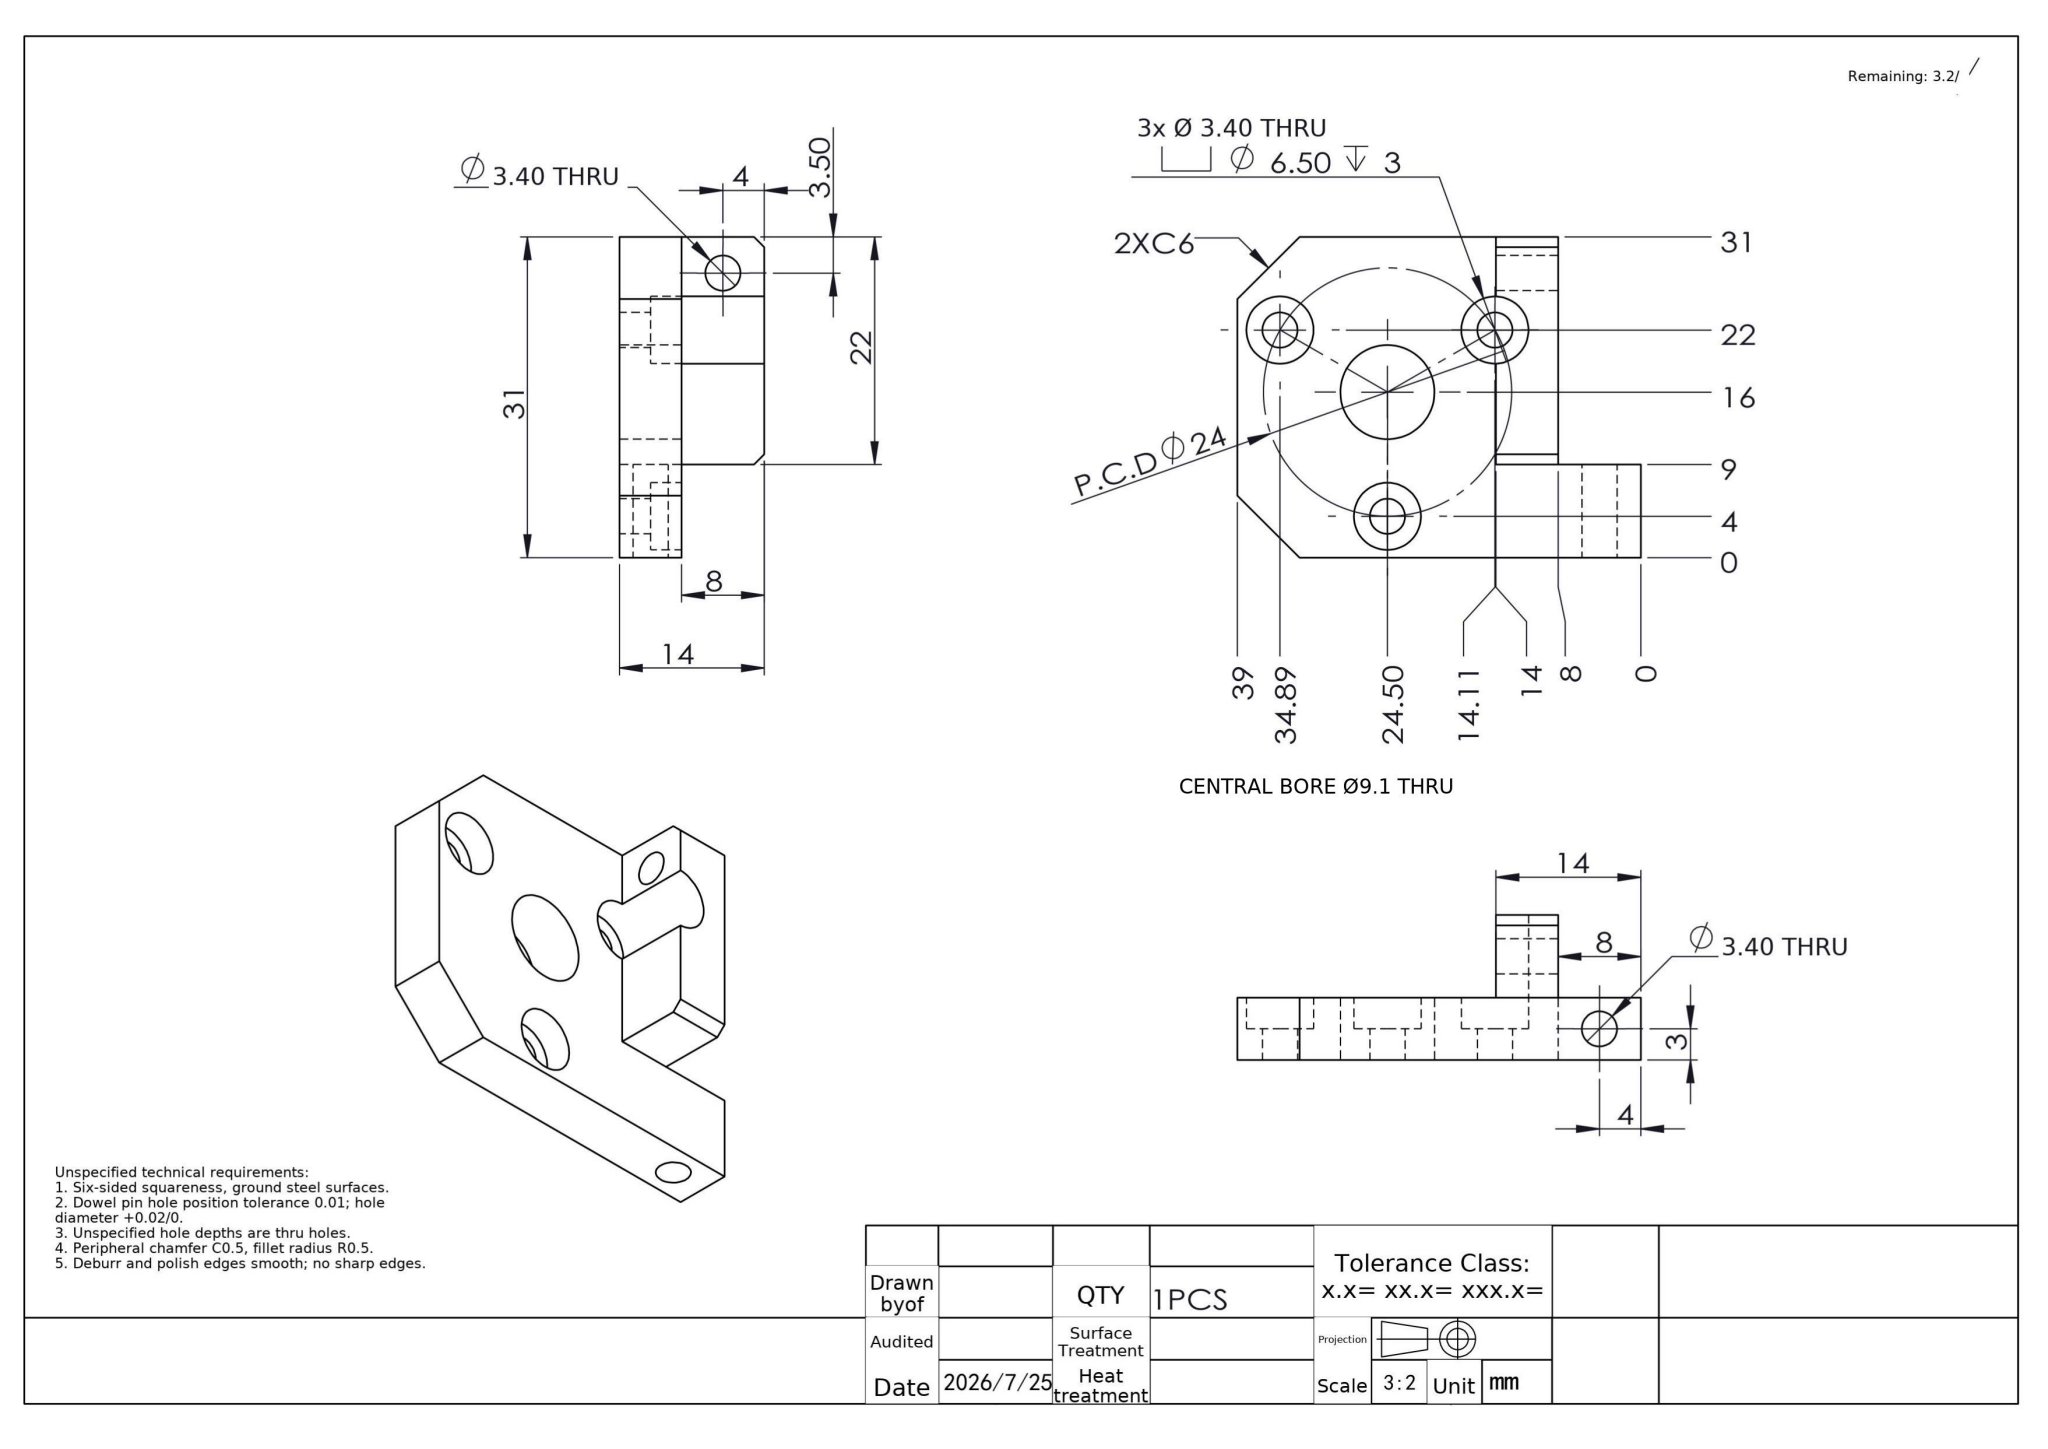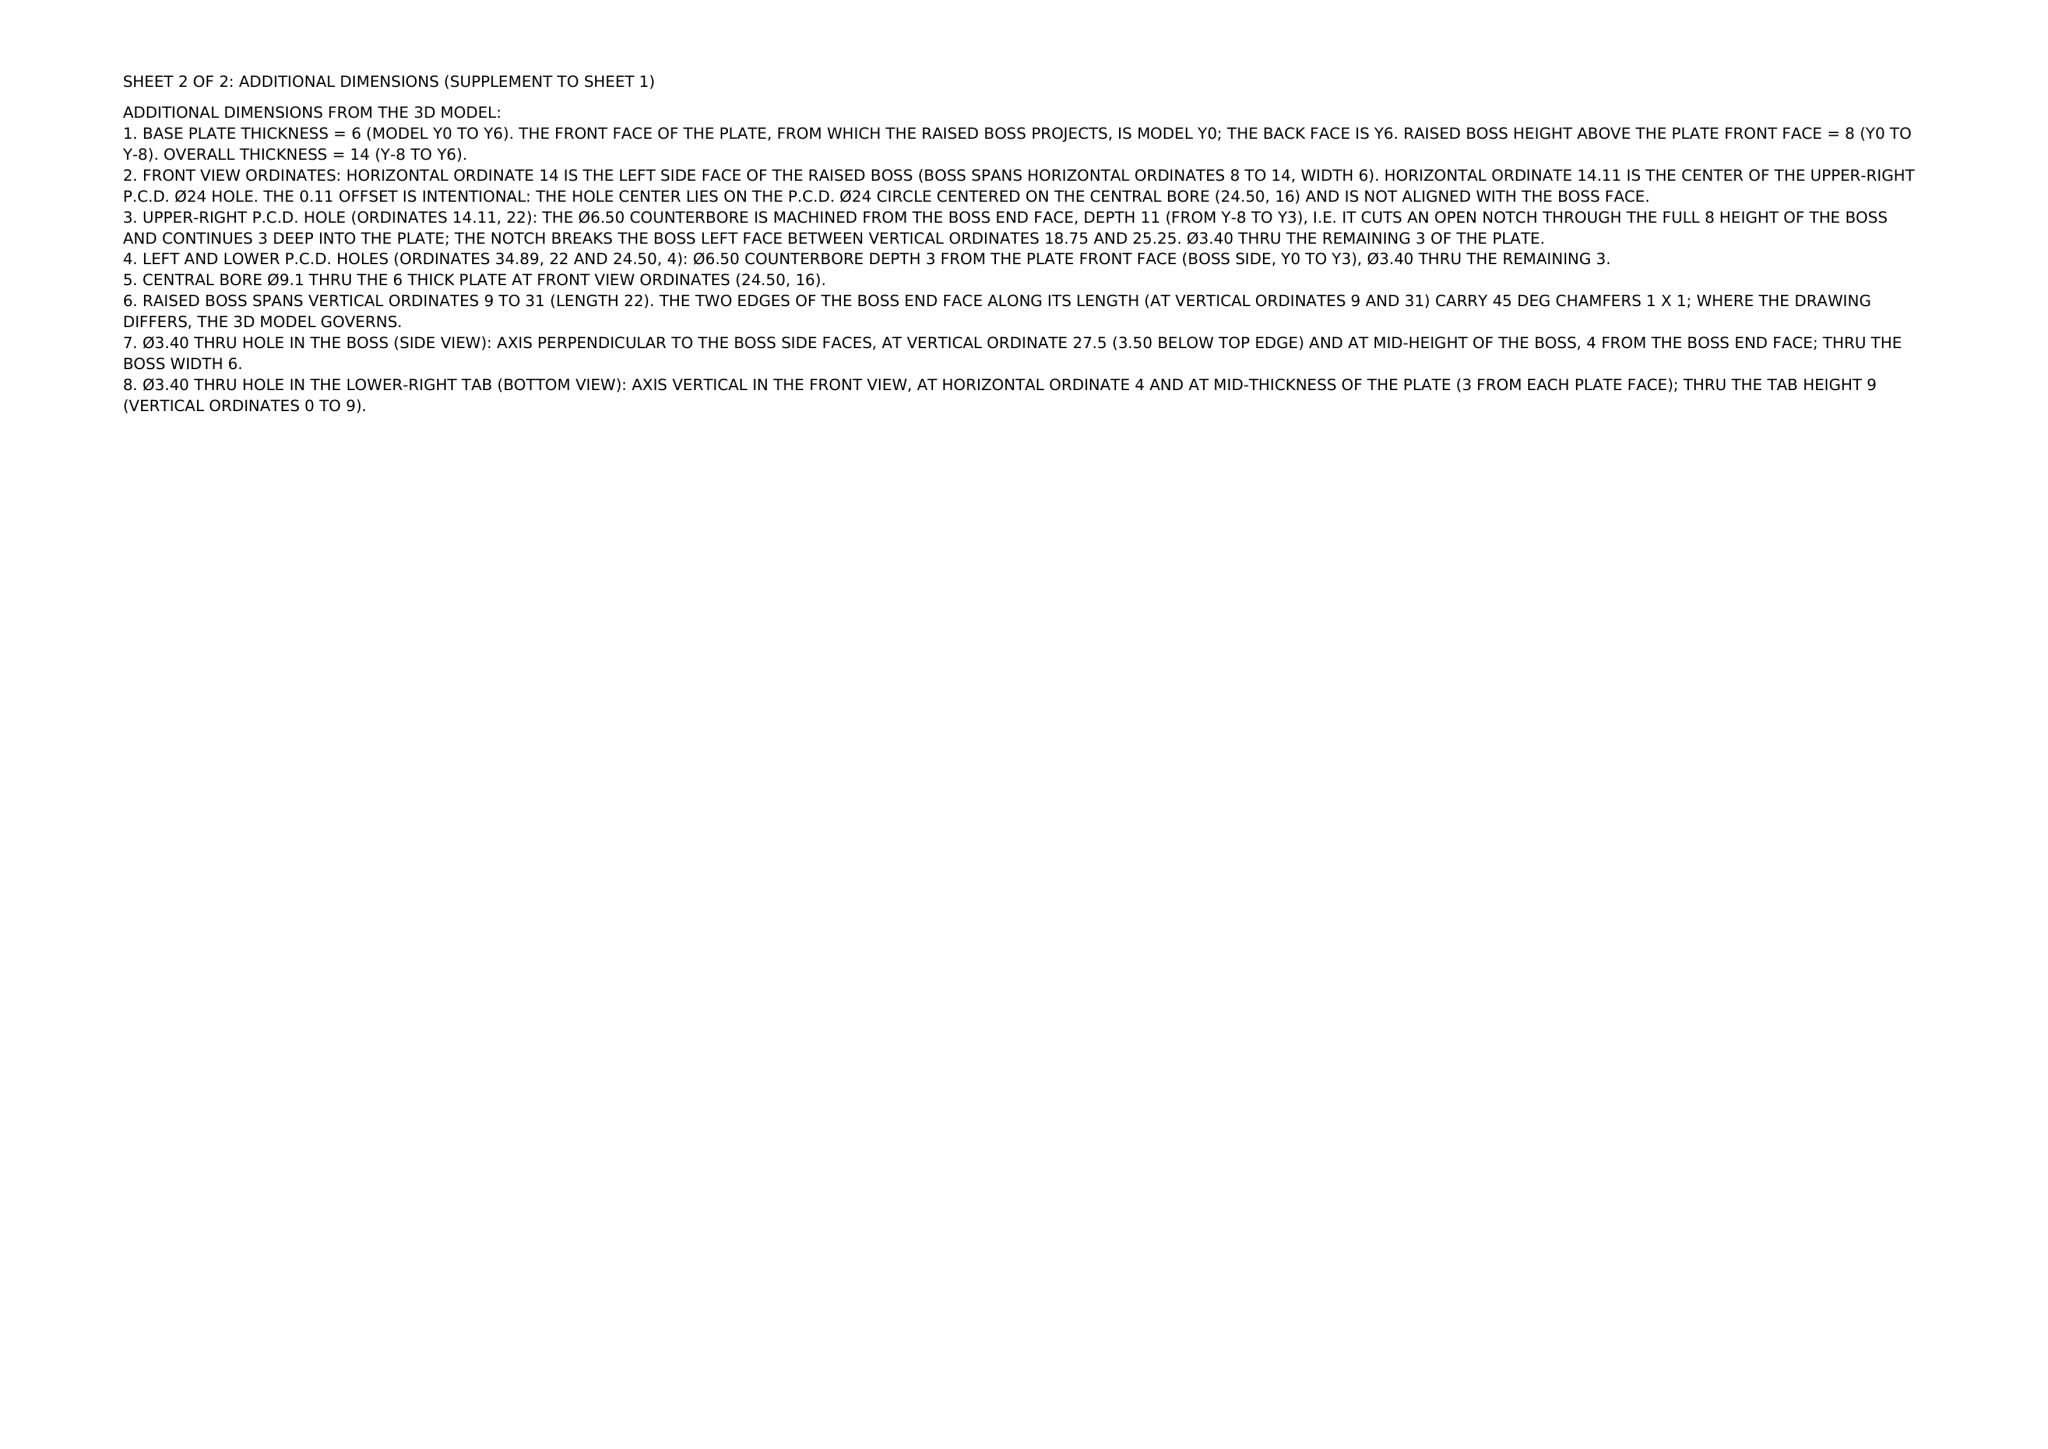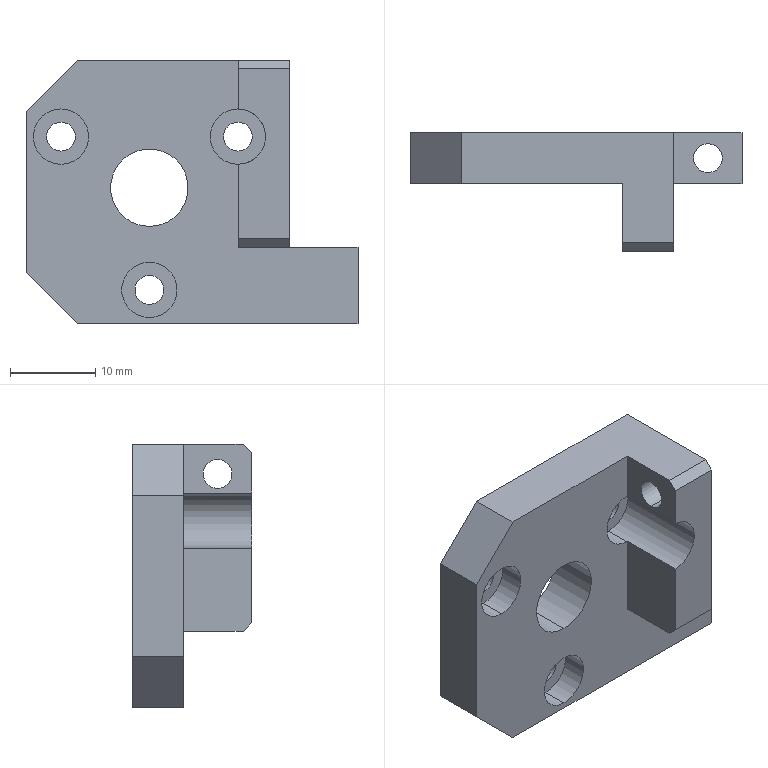Part | NX | mm | Right-Angle Dual-Tab Flanged Bore Bracket | 1 solid | 37 faces | box 39 x 14 x 31 mm | volume 5998 mm3 | plane 19 | cylinder 18 | commonest cylinder face diameters 3.4 x10 6.5 x6 9.1 x2